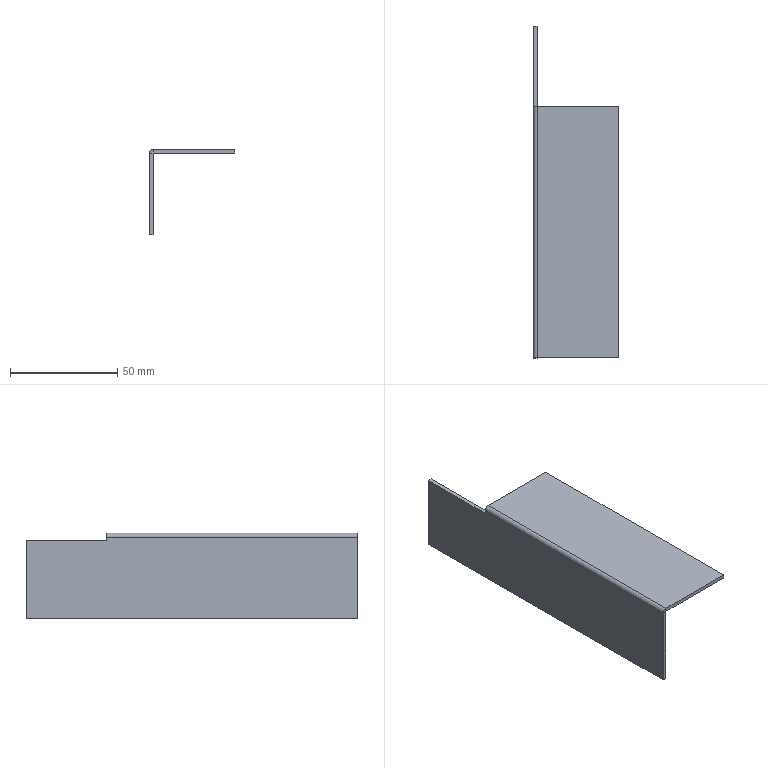Component | SolidWorks | CabinetWelding-1_ConnectingAngleIronSymmetric-1 | 1 solid | 16 faces | box 40 x 155 x 40 mm | volume 18912 mm3 | plane 14 | cylinder 2 | commonest cylinder face diameters 3.8 x1 0.2 x1
STEP:
#1=COLOUR_RGB('',0.7922,0.8196,0.9333);
#2=FILL_AREA_STYLE_COLOUR('',#1);
#3=FILL_AREA_STYLE('',(#2));
#4=SURFACE_STYLE_FILL_AREA(#3);
#5=SURFACE_SIDE_STYLE('',(#4));
#6=SURFACE_STYLE_USAGE(.BOTH.,#5);
#7=PRESENTATION_STYLE_ASSIGNMENT((#6));
#8=CARTESIAN_POINT('',(18.747,33.519,96.272));
#9=VERTEX_POINT('',#8);
#10=CARTESIAN_POINT('',(18.747,34.995,96.272));
#11=VERTEX_POINT('',#10);
#12=CARTESIAN_POINT('',(18.747,32.65,96.272));
#13=DIRECTION('',(0.,1.,0.));
#14=VECTOR('',#13,39.37);
#15=LINE('',#12,#14);
#16=EDGE_CURVE('',#9,#11,#15,.T.);
#17=ORIENTED_EDGE('',*,*,#16,.T.);
#18=CARTESIAN_POINT('',(18.747,34.995,94.835));
#19=VERTEX_POINT('',#18);
#20=CARTESIAN_POINT('',(18.747,34.995,96.41));
#21=DIRECTION('',(0.,-0.,1.));
#22=VECTOR('',#21,39.37);
#23=LINE('',#20,#22);
#24=EDGE_CURVE('',#19,#11,#23,.T.);
#25=ORIENTED_EDGE('',*,*,#24,.F.);
#26=CARTESIAN_POINT('',(18.747,28.893,94.835));
#27=VERTEX_POINT('',#26);
#28=CARTESIAN_POINT('',(18.747,28.893,94.835));
#29=DIRECTION('',(0.,1.,0.));
#30=VECTOR('',#29,39.37);
#31=LINE('',#28,#30);
#32=EDGE_CURVE('',#27,#19,#31,.T.);
#33=ORIENTED_EDGE('',*,*,#32,.F.);
#34=CARTESIAN_POINT('',(18.747,28.893,96.335));
#35=VERTEX_POINT('',#34);
#36=CARTESIAN_POINT('',(18.747,28.893,96.41));
#37=DIRECTION('',(-0.,0.,-1.));
#38=VECTOR('',#37,39.37);
#39=LINE('',#36,#38);
#40=EDGE_CURVE('',#35,#27,#39,.T.);
#41=ORIENTED_EDGE('',*,*,#40,.F.);
#42=CARTESIAN_POINT('',(18.747,33.519,96.335));
#43=VERTEX_POINT('',#42);
#44=CARTESIAN_POINT('',(18.747,28.893,96.335));
#45=DIRECTION('',(0.,1.,0.));
#46=VECTOR('',#45,39.37);
#47=LINE('',#44,#46);
#48=EDGE_CURVE('',#35,#43,#47,.T.);
#49=ORIENTED_EDGE('',*,*,#48,.T.);
#50=CARTESIAN_POINT('',(18.747,33.519,95.462));
#51=DIRECTION('',(0.,-0.,1.));
#52=VECTOR('',#51,39.37);
#53=LINE('',#50,#52);
#54=EDGE_CURVE('',#9,#43,#53,.T.);
#55=ORIENTED_EDGE('',*,*,#54,.F.);
#56=EDGE_LOOP('',(#17,#25,#33,#41,#49,#55));
#57=FACE_OUTER_BOUND('',#56,.T.);
#58=CARTESIAN_POINT('',(18.747,32.65,95.462));
#59=DIRECTION('',(1.,-0.,-0.));
#60=DIRECTION('',(0.,1.,0.));
#61=AXIS2_PLACEMENT_3D('',#58,#59,#60);
#62=PLANE('',#61);
#63=ADVANCED_FACE('',(#57),#62,.F.);
#64=CARTESIAN_POINT('',(18.818,34.995,94.835));
#65=VERTEX_POINT('',#64);
#66=CARTESIAN_POINT('',(18.818,34.995,96.272));
#67=VERTEX_POINT('',#66);
#68=CARTESIAN_POINT('',(18.818,34.995,96.41));
#69=DIRECTION('',(0.,-0.,1.));
#70=VECTOR('',#69,39.37);
#71=LINE('',#68,#70);
#72=EDGE_CURVE('',#65,#67,#71,.T.);
#73=ORIENTED_EDGE('',*,*,#72,.T.);
#74=CARTESIAN_POINT('',(18.818,33.519,96.272));
#75=VERTEX_POINT('',#74);
#76=CARTESIAN_POINT('',(18.818,32.65,96.272));
#77=DIRECTION('',(0.,1.,0.));
#78=VECTOR('',#77,39.37);
#79=LINE('',#76,#78);
#80=EDGE_CURVE('',#75,#67,#79,.T.);
#81=ORIENTED_EDGE('',*,*,#80,.F.);
#82=CARTESIAN_POINT('',(18.818,33.519,96.335));
#83=VERTEX_POINT('',#82);
#84=CARTESIAN_POINT('',(18.818,33.519,96.335));
#85=DIRECTION('',(-0.,0.,-1.));
#86=VECTOR('',#85,39.37);
#87=LINE('',#84,#86);
#88=EDGE_CURVE('',#83,#75,#87,.T.);
#89=ORIENTED_EDGE('',*,*,#88,.F.);
#90=CARTESIAN_POINT('',(18.818,28.893,96.335));
#91=VERTEX_POINT('',#90);
#92=CARTESIAN_POINT('',(18.818,28.893,96.335));
#93=DIRECTION('',(0.,1.,0.));
#94=VECTOR('',#93,39.37);
#95=LINE('',#92,#94);
#96=EDGE_CURVE('',#91,#83,#95,.T.);
#97=ORIENTED_EDGE('',*,*,#96,.F.);
#98=CARTESIAN_POINT('',(18.818,28.893,94.835));
#99=VERTEX_POINT('',#98);
#100=CARTESIAN_POINT('',(18.818,28.893,96.41));
#101=DIRECTION('',(-0.,0.,-1.));
#102=VECTOR('',#101,39.37);
#103=LINE('',#100,#102);
#104=EDGE_CURVE('',#91,#99,#103,.T.);
#105=ORIENTED_EDGE('',*,*,#104,.T.);
#106=CARTESIAN_POINT('',(18.818,28.893,94.835));
#107=DIRECTION('',(0.,1.,0.));
#108=VECTOR('',#107,39.37);
#109=LINE('',#106,#108);
#110=EDGE_CURVE('',#99,#65,#109,.T.);
#111=ORIENTED_EDGE('',*,*,#110,.T.);
#112=EDGE_LOOP('',(#73,#81,#89,#97,#105,#111));
#113=FACE_OUTER_BOUND('',#112,.T.);
#114=CARTESIAN_POINT('',(18.818,32.65,95.462));
#115=DIRECTION('',(1.,-0.,-0.));
#116=DIRECTION('',(0.,1.,0.));
#117=AXIS2_PLACEMENT_3D('',#114,#115,#116);
#118=PLANE('',#117);
#119=ADVANCED_FACE('',(#113),#118,.T.);
#120=ORIENTED_EDGE('',*,*,#24,.T.);
#121=CARTESIAN_POINT('',(18.747,34.995,96.272));
#122=DIRECTION('',(1.,-0.,-0.));
#123=VECTOR('',#122,39.37);
#124=LINE('',#121,#123);
#125=EDGE_CURVE('',#11,#67,#124,.T.);
#126=ORIENTED_EDGE('',*,*,#125,.T.);
#127=ORIENTED_EDGE('',*,*,#72,.F.);
#128=CARTESIAN_POINT('',(18.747,34.995,94.835));
#129=DIRECTION('',(1.,-0.,-0.));
#130=VECTOR('',#129,39.37);
#131=LINE('',#128,#130);
#132=EDGE_CURVE('',#19,#65,#131,.T.);
#133=ORIENTED_EDGE('',*,*,#132,.F.);
#134=EDGE_LOOP('',(#120,#126,#127,#133));
#135=FACE_OUTER_BOUND('',#134,.T.);
#136=CARTESIAN_POINT('',(18.747,34.995,96.41));
#137=DIRECTION('',(0.,1.,0.));
#138=DIRECTION('',(0.,-0.,1.));
#139=AXIS2_PLACEMENT_3D('',#136,#137,#138);
#140=PLANE('',#139);
#141=ADVANCED_FACE('',(#135),#140,.T.);
#142=ORIENTED_EDGE('',*,*,#104,.F.);
#143=CARTESIAN_POINT('',(18.818,28.893,96.335));
#144=DIRECTION('',(-1.,0.,0.));
#145=VECTOR('',#144,39.37);
#146=LINE('',#143,#145);
#147=EDGE_CURVE('',#91,#35,#146,.T.);
#148=ORIENTED_EDGE('',*,*,#147,.T.);
#149=ORIENTED_EDGE('',*,*,#40,.T.);
#150=CARTESIAN_POINT('',(18.747,28.893,94.835));
#151=DIRECTION('',(1.,-0.,-0.));
#152=VECTOR('',#151,39.37);
#153=LINE('',#150,#152);
#154=EDGE_CURVE('',#27,#99,#153,.T.);
#155=ORIENTED_EDGE('',*,*,#154,.T.);
#156=EDGE_LOOP('',(#142,#148,#149,#155));
#157=FACE_OUTER_BOUND('',#156,.T.);
#158=CARTESIAN_POINT('',(18.747,28.893,96.41));
#159=DIRECTION('',(-0.,-1.,-0.));
#160=DIRECTION('',(1.,-0.,-0.));
#161=AXIS2_PLACEMENT_3D('',#158,#159,#160);
#162=PLANE('',#161);
#163=ADVANCED_FACE('',(#157),#162,.T.);
#164=ORIENTED_EDGE('',*,*,#110,.F.);
#165=ORIENTED_EDGE('',*,*,#154,.F.);
#166=ORIENTED_EDGE('',*,*,#32,.T.);
#167=ORIENTED_EDGE('',*,*,#132,.T.);
#168=EDGE_LOOP('',(#164,#165,#166,#167));
#169=FACE_OUTER_BOUND('',#168,.T.);
#170=CARTESIAN_POINT('',(18.747,28.893,94.835));
#171=DIRECTION('',(-0.,0.,-1.));
#172=DIRECTION('',(-1.,0.,0.));
#173=AXIS2_PLACEMENT_3D('',#170,#171,#172);
#174=PLANE('',#173);
#175=ADVANCED_FACE('',(#169),#174,.T.);
#176=ORIENTED_EDGE('',*,*,#88,.T.);
#177=CARTESIAN_POINT('',(18.747,33.519,96.272));
#178=DIRECTION('',(1.,-0.,-0.));
#179=VECTOR('',#178,39.37);
#180=LINE('',#177,#179);
#181=EDGE_CURVE('',#9,#75,#180,.T.);
#182=ORIENTED_EDGE('',*,*,#181,.F.);
#183=ORIENTED_EDGE('',*,*,#54,.T.);
#184=CARTESIAN_POINT('',(18.818,33.519,96.335));
#185=DIRECTION('',(-1.,0.,0.));
#186=VECTOR('',#185,39.37);
#187=LINE('',#184,#186);
#188=EDGE_CURVE('',#83,#43,#187,.T.);
#189=ORIENTED_EDGE('',*,*,#188,.F.);
#190=EDGE_LOOP('',(#176,#182,#183,#189));
#191=FACE_OUTER_BOUND('',#190,.T.);
#192=CARTESIAN_POINT('',(18.818,33.519,96.335));
#193=DIRECTION('',(0.,1.,0.));
#194=DIRECTION('',(-1.,0.,0.));
#195=AXIS2_PLACEMENT_3D('',#192,#193,#194);
#196=PLANE('',#195);
#197=ADVANCED_FACE('',(#191),#196,.T.);
#198=CARTESIAN_POINT('',(18.822,33.519,96.339));
#199=VERTEX_POINT('',#198);
#200=CARTESIAN_POINT('',(18.822,33.519,96.41));
#201=VERTEX_POINT('',#200);
#202=CARTESIAN_POINT('',(18.822,33.519,96.41));
#203=DIRECTION('',(-0.,-0.,1.));
#204=VECTOR('',#203,39.37);
#205=LINE('',#202,#204);
#206=EDGE_CURVE('',#199,#201,#205,.T.);
#207=ORIENTED_EDGE('',*,*,#206,.F.);
#208=CARTESIAN_POINT('',(18.822,33.519,96.335));
#209=DIRECTION('',(0.,1.,0.));
#210=DIRECTION('',(1.,0.,0.));
#211=AXIS2_PLACEMENT_3D('',#208,#209,#210);
#212=CIRCLE('',#211,0.003937);
#213=EDGE_CURVE('',#83,#199,#212,.T.);
#214=ORIENTED_EDGE('',*,*,#213,.F.);
#215=ORIENTED_EDGE('',*,*,#188,.T.);
#216=CARTESIAN_POINT('',(18.822,33.519,96.335));
#217=DIRECTION('',(0.,1.,0.));
#218=DIRECTION('',(1.,0.,0.));
#219=AXIS2_PLACEMENT_3D('',#216,#217,#218);
#220=CIRCLE('',#219,0.0748);
#221=EDGE_CURVE('',#43,#201,#220,.T.);
#222=ORIENTED_EDGE('',*,*,#221,.T.);
#223=EDGE_LOOP('',(#207,#214,#215,#222));
#224=FACE_OUTER_BOUND('',#223,.T.);
#225=CARTESIAN_POINT('',(18.822,33.519,96.335));
#226=DIRECTION('',(0.,1.,0.));
#227=DIRECTION('',(-1.,0.,0.));
#228=AXIS2_PLACEMENT_3D('',#225,#226,#227);
#229=PLANE('',#228);
#230=ADVANCED_FACE('',(#224),#229,.T.);
#231=CARTESIAN_POINT('',(18.822,28.893,96.339));
#232=VERTEX_POINT('',#231);
#233=CARTESIAN_POINT('',(18.822,28.893,96.335));
#234=DIRECTION('',(-0.,-1.,-0.));
#235=DIRECTION('',(1.,0.,0.));
#236=AXIS2_PLACEMENT_3D('',#233,#234,#235);
#237=CIRCLE('',#236,0.003937);
#238=EDGE_CURVE('',#232,#91,#237,.T.);
#239=ORIENTED_EDGE('',*,*,#238,.F.);
#240=CARTESIAN_POINT('',(18.822,28.893,96.41));
#241=VERTEX_POINT('',#240);
#242=CARTESIAN_POINT('',(18.822,28.893,96.339));
#243=DIRECTION('',(-0.,-0.,1.));
#244=VECTOR('',#243,39.37);
#245=LINE('',#242,#244);
#246=EDGE_CURVE('',#232,#241,#245,.T.);
#247=ORIENTED_EDGE('',*,*,#246,.T.);
#248=CARTESIAN_POINT('',(18.822,28.893,96.335));
#249=DIRECTION('',(-0.,-1.,-0.));
#250=DIRECTION('',(1.,0.,0.));
#251=AXIS2_PLACEMENT_3D('',#248,#249,#250);
#252=CIRCLE('',#251,0.0748);
#253=EDGE_CURVE('',#241,#35,#252,.T.);
#254=ORIENTED_EDGE('',*,*,#253,.T.);
#255=ORIENTED_EDGE('',*,*,#147,.F.);
#256=EDGE_LOOP('',(#239,#247,#254,#255));
#257=FACE_OUTER_BOUND('',#256,.T.);
#258=CARTESIAN_POINT('',(18.822,28.893,96.335));
#259=DIRECTION('',(0.,1.,0.));
#260=DIRECTION('',(-1.,0.,0.));
#261=AXIS2_PLACEMENT_3D('',#258,#259,#260);
#262=PLANE('',#261);
#263=ADVANCED_FACE('',(#257),#262,.F.);
#264=ORIENTED_EDGE('',*,*,#48,.F.);
#265=ORIENTED_EDGE('',*,*,#253,.F.);
#266=CARTESIAN_POINT('',(18.822,32.65,96.41));
#267=DIRECTION('',(-0.,-1.,-0.));
#268=VECTOR('',#267,39.37);
#269=LINE('',#266,#268);
#270=EDGE_CURVE('',#201,#241,#269,.T.);
#271=ORIENTED_EDGE('',*,*,#270,.F.);
#272=ORIENTED_EDGE('',*,*,#221,.F.);
#273=EDGE_LOOP('',(#264,#265,#271,#272));
#274=FACE_OUTER_BOUND('',#273,.T.);
#275=CARTESIAN_POINT('',(18.822,28.893,96.335));
#276=DIRECTION('',(-0.,-1.,-0.));
#277=DIRECTION('',(0.,0.,1.));
#278=AXIS2_PLACEMENT_3D('',#275,#276,#277);
#279=CYLINDRICAL_SURFACE('',#278,0.0748);
#280=ADVANCED_FACE('',(#274),#279,.T.);
#281=ORIENTED_EDGE('',*,*,#96,.T.);
#282=ORIENTED_EDGE('',*,*,#213,.T.);
#283=CARTESIAN_POINT('',(18.822,33.519,96.339));
#284=DIRECTION('',(-0.,-1.,-0.));
#285=VECTOR('',#284,39.37);
#286=LINE('',#283,#285);
#287=EDGE_CURVE('',#199,#232,#286,.T.);
#288=ORIENTED_EDGE('',*,*,#287,.T.);
#289=ORIENTED_EDGE('',*,*,#238,.T.);
#290=EDGE_LOOP('',(#281,#282,#288,#289));
#291=FACE_OUTER_BOUND('',#290,.T.);
#292=CARTESIAN_POINT('',(18.822,28.893,96.335));
#293=DIRECTION('',(-0.,-1.,-0.));
#294=DIRECTION('',(0.,0.,1.));
#295=AXIS2_PLACEMENT_3D('',#292,#293,#294);
#296=CYLINDRICAL_SURFACE('',#295,0.003937);
#297=ADVANCED_FACE('',(#291),#296,.F.);
#298=CARTESIAN_POINT('',(20.322,28.893,96.41));
#299=VERTEX_POINT('',#298);
#300=CARTESIAN_POINT('',(18.818,28.893,96.41));
#301=DIRECTION('',(-1.,0.,-0.));
#302=VECTOR('',#301,39.37);
#303=LINE('',#300,#302);
#304=EDGE_CURVE('',#299,#241,#303,.T.);
#305=ORIENTED_EDGE('',*,*,#304,.T.);
#306=ORIENTED_EDGE('',*,*,#246,.F.);
#307=CARTESIAN_POINT('',(20.322,28.893,96.339));
#308=VERTEX_POINT('',#307);
#309=CARTESIAN_POINT('',(18.818,28.893,96.339));
#310=DIRECTION('',(-1.,0.,-0.));
#311=VECTOR('',#310,39.37);
#312=LINE('',#309,#311);
#313=EDGE_CURVE('',#308,#232,#312,.T.);
#314=ORIENTED_EDGE('',*,*,#313,.F.);
#315=CARTESIAN_POINT('',(20.322,28.893,96.41));
#316=DIRECTION('',(0.,0.,-1.));
#317=VECTOR('',#316,39.37);
#318=LINE('',#315,#317);
#319=EDGE_CURVE('',#299,#308,#318,.T.);
#320=ORIENTED_EDGE('',*,*,#319,.F.);
#321=EDGE_LOOP('',(#305,#306,#314,#320));
#322=FACE_OUTER_BOUND('',#321,.T.);
#323=CARTESIAN_POINT('',(18.818,28.893,96.41));
#324=DIRECTION('',(-0.,-1.,-0.));
#325=DIRECTION('',(1.,-0.,-0.));
#326=AXIS2_PLACEMENT_3D('',#323,#324,#325);
#327=PLANE('',#326);
#328=ADVANCED_FACE('',(#322),#327,.T.);
#329=CARTESIAN_POINT('',(20.322,33.519,96.339));
#330=VERTEX_POINT('',#329);
#331=CARTESIAN_POINT('',(18.818,33.519,96.339));
#332=DIRECTION('',(1.,-0.,0.));
#333=VECTOR('',#332,39.37);
#334=LINE('',#331,#333);
#335=EDGE_CURVE('',#199,#330,#334,.T.);
#336=ORIENTED_EDGE('',*,*,#335,.F.);
#337=ORIENTED_EDGE('',*,*,#206,.T.);
#338=CARTESIAN_POINT('',(20.322,33.519,96.41));
#339=VERTEX_POINT('',#338);
#340=CARTESIAN_POINT('',(20.322,33.519,96.41));
#341=DIRECTION('',(1.,-0.,0.));
#342=VECTOR('',#341,39.37);
#343=LINE('',#340,#342);
#344=EDGE_CURVE('',#201,#339,#343,.T.);
#345=ORIENTED_EDGE('',*,*,#344,.T.);
#346=CARTESIAN_POINT('',(20.322,33.519,96.41));
#347=DIRECTION('',(0.,0.,-1.));
#348=VECTOR('',#347,39.37);
#349=LINE('',#346,#348);
#350=EDGE_CURVE('',#339,#330,#349,.T.);
#351=ORIENTED_EDGE('',*,*,#350,.T.);
#352=EDGE_LOOP('',(#336,#337,#345,#351));
#353=FACE_OUTER_BOUND('',#352,.T.);
#354=CARTESIAN_POINT('',(20.322,33.519,96.41));
#355=DIRECTION('',(0.,1.,0.));
#356=DIRECTION('',(-1.,0.,0.));
#357=AXIS2_PLACEMENT_3D('',#354,#355,#356);
#358=PLANE('',#357);
#359=ADVANCED_FACE('',(#353),#358,.T.);
#360=ORIENTED_EDGE('',*,*,#344,.F.);
#361=ORIENTED_EDGE('',*,*,#270,.T.);
#362=ORIENTED_EDGE('',*,*,#304,.F.);
#363=CARTESIAN_POINT('',(20.322,28.893,96.41));
#364=DIRECTION('',(-0.,-1.,-0.));
#365=VECTOR('',#364,39.37);
#366=LINE('',#363,#365);
#367=EDGE_CURVE('',#339,#299,#366,.T.);
#368=ORIENTED_EDGE('',*,*,#367,.F.);
#369=EDGE_LOOP('',(#360,#361,#362,#368));
#370=FACE_OUTER_BOUND('',#369,.T.);
#371=CARTESIAN_POINT('',(18.818,32.65,96.41));
#372=DIRECTION('',(-0.,-0.,1.));
#373=DIRECTION('',(1.,-0.,0.));
#374=AXIS2_PLACEMENT_3D('',#371,#372,#373);
#375=PLANE('',#374);
#376=ADVANCED_FACE('',(#370),#375,.T.);
#377=ORIENTED_EDGE('',*,*,#287,.F.);
#378=ORIENTED_EDGE('',*,*,#335,.T.);
#379=CARTESIAN_POINT('',(20.322,32.65,96.339));
#380=DIRECTION('',(-0.,-1.,-0.));
#381=VECTOR('',#380,39.37);
#382=LINE('',#379,#381);
#383=EDGE_CURVE('',#330,#308,#382,.T.);
#384=ORIENTED_EDGE('',*,*,#383,.T.);
#385=ORIENTED_EDGE('',*,*,#313,.T.);
#386=EDGE_LOOP('',(#377,#378,#384,#385));
#387=FACE_OUTER_BOUND('',#386,.T.);
#388=CARTESIAN_POINT('',(18.818,32.65,96.339));
#389=DIRECTION('',(-0.,-0.,1.));
#390=DIRECTION('',(1.,-0.,0.));
#391=AXIS2_PLACEMENT_3D('',#388,#389,#390);
#392=PLANE('',#391);
#393=ADVANCED_FACE('',(#387),#392,.F.);
#394=ORIENTED_EDGE('',*,*,#383,.F.);
#395=ORIENTED_EDGE('',*,*,#350,.F.);
#396=ORIENTED_EDGE('',*,*,#367,.T.);
#397=ORIENTED_EDGE('',*,*,#319,.T.);
#398=EDGE_LOOP('',(#394,#395,#396,#397));
#399=FACE_OUTER_BOUND('',#398,.T.);
#400=CARTESIAN_POINT('',(20.322,28.893,96.41));
#401=DIRECTION('',(1.,-0.,0.));
#402=DIRECTION('',(0.,0.,-1.));
#403=AXIS2_PLACEMENT_3D('',#400,#401,#402);
#404=PLANE('',#403);
#405=ADVANCED_FACE('',(#399),#404,.T.);
#406=ORIENTED_EDGE('',*,*,#125,.F.);
#407=ORIENTED_EDGE('',*,*,#16,.F.);
#408=ORIENTED_EDGE('',*,*,#181,.T.);
#409=ORIENTED_EDGE('',*,*,#80,.T.);
#410=EDGE_LOOP('',(#406,#407,#408,#409));
#411=FACE_OUTER_BOUND('',#410,.T.);
#412=CARTESIAN_POINT('',(18.747,32.65,96.272));
#413=DIRECTION('',(-0.,0.,-1.));
#414=DIRECTION('',(0.,1.,0.));
#415=AXIS2_PLACEMENT_3D('',#412,#413,#414);
#416=PLANE('',#415);
#417=ADVANCED_FACE('',(#411),#416,.F.);
#418=CLOSED_SHELL('',(#63,#119,#141,#163,#175,#197,#230,#263,#280,#297,#328,#359,#376,#393,#405,#417));
#419=MANIFOLD_SOLID_BREP('',#418);
#420=STYLED_ITEM('',(#7),#419);
#421=(LENGTH_UNIT()NAMED_UNIT(*)SI_UNIT($,.METRE.));
#422=LENGTH_MEASURE_WITH_UNIT(LENGTH_MEASURE(0.0254),#421);
#423=DIMENSIONAL_EXPONENTS(1.,0.,0.,0.,0.,0.,0.);
#424=(CONVERSION_BASED_UNIT('',#422)LENGTH_UNIT()NAMED_UNIT(#423));
#425=UNCERTAINTY_MEASURE_WITH_UNIT(LENGTH_MEASURE(0.00001),#424,'','');
#426=(NAMED_UNIT(*)PLANE_ANGLE_UNIT()SI_UNIT($,.RADIAN.));
#427=(NAMED_UNIT(*)SI_UNIT($,.STERADIAN.)SOLID_ANGLE_UNIT());
#428=(GEOMETRIC_REPRESENTATION_CONTEXT(3)GLOBAL_UNCERTAINTY_ASSIGNED_CONTEXT((#425))GLOBAL_UNIT_ASSIGNED_CONTEXT((#424,#426,#427))REPRESENTATION_CONTEXT('',''));
#429=MECHANICAL_DESIGN_GEOMETRIC_PRESENTATION_REPRESENTATION('',(#420),#428);
#430=CARTESIAN_POINT('',(0.,0.,0.));
#431=DIRECTION('',(0.,0.,1.));
#432=DIRECTION('',(1.,0.,0.));
#433=AXIS2_PLACEMENT_3D('',#430,#431,#432);
#434=(LENGTH_UNIT()NAMED_UNIT(*)SI_UNIT($,.METRE.));
#435=LENGTH_MEASURE_WITH_UNIT(LENGTH_MEASURE(0.0254),#434);
#436=DIMENSIONAL_EXPONENTS(1.,0.,0.,0.,0.,0.,0.);
#437=(CONVERSION_BASED_UNIT('',#435)LENGTH_UNIT()NAMED_UNIT(#436));
#438=UNCERTAINTY_MEASURE_WITH_UNIT(LENGTH_MEASURE(0.00001),#437,'','');
#439=(NAMED_UNIT(*)PLANE_ANGLE_UNIT()SI_UNIT($,.RADIAN.));
#440=(NAMED_UNIT(*)SI_UNIT($,.STERADIAN.)SOLID_ANGLE_UNIT());
#441=(GEOMETRIC_REPRESENTATION_CONTEXT(3)GLOBAL_UNCERTAINTY_ASSIGNED_CONTEXT((#438))GLOBAL_UNIT_ASSIGNED_CONTEXT((#437,#439,#440))REPRESENTATION_CONTEXT('',''));
#442=ADVANCED_BREP_SHAPE_REPRESENTATION('',(#419,#433),#441);
#443=PRESENTATION_LAYER_ASSIGNMENT('','',(#420));